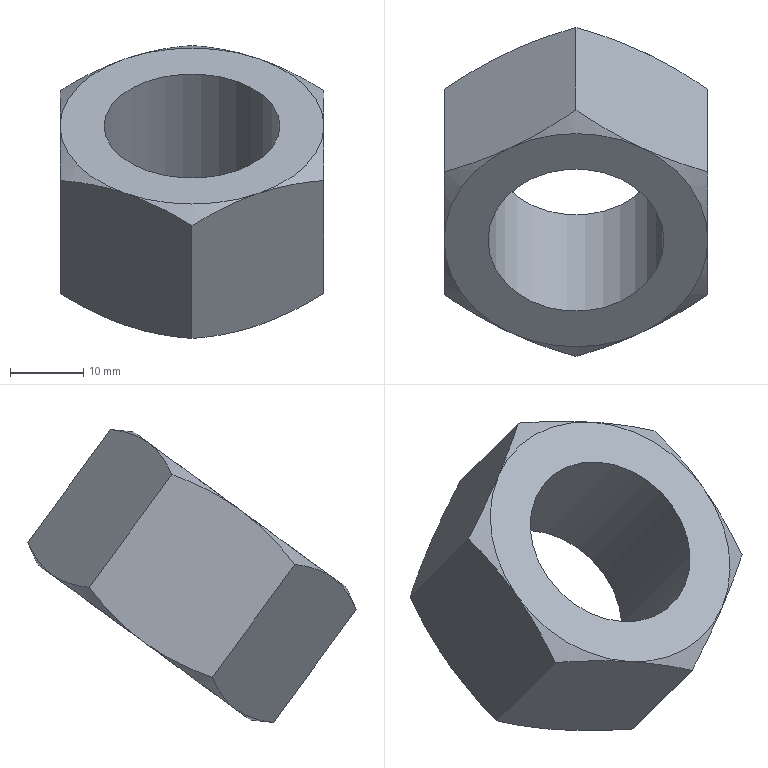Component | SolidWorks | hex nut gradec_iso-10 | 1 solid | 22 faces | box 36 x 44.81 x 39.96 mm | volume 14839 mm3 | cone 12 | plane 8 | cylinder 2 | commonest cylinder face diameters 24 x2
STEP:
#1=COLOUR_RGB('',0.7922,0.8196,0.9333);
#2=FILL_AREA_STYLE_COLOUR('',#1);
#3=FILL_AREA_STYLE('',(#2));
#4=SURFACE_STYLE_FILL_AREA(#3);
#5=SURFACE_SIDE_STYLE('',(#4));
#6=SURFACE_STYLE_USAGE(.BOTH.,#5);
#7=PRESENTATION_STYLE_ASSIGNMENT((#6));
#8=CARTESIAN_POINT('',(-39.394,24.717,14.549));
#9=VERTEX_POINT('',#8);
#10=CARTESIAN_POINT('',(-38.449,24.717,14.549));
#11=VERTEX_POINT('',#10);
#12=CARTESIAN_POINT('',(-38.921,24.717,14.549));
#13=DIRECTION('',(0.,-0.5907,0.8069));
#14=DIRECTION('',(1.,0.,0.));
#15=AXIS2_PLACEMENT_3D('',#12,#13,#14);
#16=CIRCLE('',#15,0.4724);
#17=EDGE_CURVE('',#9,#11,#16,.T.);
#18=ORIENTED_EDGE('',*,*,#17,.F.);
#19=CARTESIAN_POINT('',(-39.394,24.198,15.258));
#20=VERTEX_POINT('',#19);
#21=CARTESIAN_POINT('',(-39.394,24.717,14.549));
#22=DIRECTION('',(0.,-0.5907,0.8069));
#23=VECTOR('',#22,39.37);
#24=LINE('',#21,#23);
#25=EDGE_CURVE('',#9,#20,#24,.T.);
#26=ORIENTED_EDGE('',*,*,#25,.T.);
#27=CARTESIAN_POINT('',(-38.449,24.198,15.258));
#28=VERTEX_POINT('',#27);
#29=CARTESIAN_POINT('',(-38.921,24.198,15.258));
#30=DIRECTION('',(0.,-0.5907,0.8069));
#31=DIRECTION('',(1.,0.,0.));
#32=AXIS2_PLACEMENT_3D('',#29,#30,#31);
#33=CIRCLE('',#32,0.4724);
#34=EDGE_CURVE('',#20,#28,#33,.T.);
#35=ORIENTED_EDGE('',*,*,#34,.T.);
#36=CARTESIAN_POINT('',(-38.449,24.717,14.549));
#37=DIRECTION('',(0.,-0.5907,0.8069));
#38=VECTOR('',#37,39.37);
#39=LINE('',#36,#38);
#40=EDGE_CURVE('',#11,#28,#39,.T.);
#41=ORIENTED_EDGE('',*,*,#40,.F.);
#42=EDGE_LOOP('',(#18,#26,#35,#41));
#43=FACE_OUTER_BOUND('',#42,.T.);
#44=CARTESIAN_POINT('',(-38.921,24.717,14.549));
#45=DIRECTION('',(0.,-0.5907,0.8069));
#46=DIRECTION('',(1.,0.,0.));
#47=AXIS2_PLACEMENT_3D('',#44,#45,#46);
#48=CYLINDRICAL_SURFACE('',#47,0.4724);
#49=ADVANCED_FACE('',(#43),#48,.F.);
#50=CARTESIAN_POINT('',(-39.63,25.01,14.842));
#51=VERTEX_POINT('',#50);
#52=CARTESIAN_POINT('',(-39.63,24.566,15.448));
#53=VERTEX_POINT('',#52);
#54=CARTESIAN_POINT('',(-39.63,25.047,14.791));
#55=DIRECTION('',(0.,-0.5907,0.8069));
#56=VECTOR('',#55,39.37);
#57=LINE('',#54,#56);
#58=EDGE_CURVE('',#51,#53,#57,.T.);
#59=ORIENTED_EDGE('',*,*,#58,.T.);
#60=CARTESIAN_POINT('',(-39.276,24.693,15.62));
#61=VERTEX_POINT('',#60);
#62=CARTESIAN_POINT('',(-39.63,24.566,15.448));
#63=CARTESIAN_POINT('',(-39.572,24.581,15.484));
#64=CARTESIAN_POINT('',(-39.514,24.599,15.517));
#65=CARTESIAN_POINT('',(-39.396,24.641,15.575));
#66=CARTESIAN_POINT('',(-39.336,24.665,15.6));
#67=CARTESIAN_POINT('',(-39.276,24.693,15.62));
#68=B_SPLINE_CURVE_WITH_KNOTS('',3,(#62,#63,#64,#65,#66,#67),.UNSPECIFIED.,.F.,.F.,(4,2,4),(0.00000024,0.005258,0.01052),.UNSPECIFIED.);
#69=EDGE_CURVE('',#53,#61,#68,.T.);
#70=ORIENTED_EDGE('',*,*,#69,.T.);
#71=CARTESIAN_POINT('',(-38.921,24.896,15.69));
#72=VERTEX_POINT('',#71);
#73=CARTESIAN_POINT('',(-39.276,24.693,15.62));
#74=CARTESIAN_POINT('',(-39.261,24.701,15.626));
#75=CARTESIAN_POINT('',(-39.245,24.708,15.63));
#76=CARTESIAN_POINT('',(-39.215,24.723,15.639));
#77=CARTESIAN_POINT('',(-39.2,24.73,15.644));
#78=CARTESIAN_POINT('',(-39.156,24.754,15.655));
#79=CARTESIAN_POINT('',(-39.126,24.77,15.662));
#80=CARTESIAN_POINT('',(-39.037,24.821,15.679));
#81=CARTESIAN_POINT('',(-38.979,24.858,15.686));
#82=CARTESIAN_POINT('',(-38.921,24.896,15.69));
#83=B_SPLINE_CURVE_WITH_KNOTS('',3,(#73,#74,#75,#76,#77,#78,#79,#80,#81,#82),.UNSPECIFIED.,.F.,.F.,(4,2,2,2,4),(0.01052,0.01183,0.01313,0.01575,0.02099),.UNSPECIFIED.);
#84=EDGE_CURVE('',#61,#72,#83,.T.);
#85=ORIENTED_EDGE('',*,*,#84,.T.);
#86=CARTESIAN_POINT('',(-38.921,25.34,15.084));
#87=VERTEX_POINT('',#86);
#88=CARTESIAN_POINT('',(-38.921,25.377,15.033));
#89=DIRECTION('',(0.,-0.5907,0.8069));
#90=VECTOR('',#89,39.37);
#91=LINE('',#88,#90);
#92=EDGE_CURVE('',#87,#72,#91,.T.);
#93=ORIENTED_EDGE('',*,*,#92,.F.);
#94=CARTESIAN_POINT('',(-39.276,25.212,14.912));
#95=VERTEX_POINT('',#94);
#96=CARTESIAN_POINT('',(-39.276,25.212,14.912));
#97=CARTESIAN_POINT('',(-39.261,25.219,14.917));
#98=CARTESIAN_POINT('',(-39.245,25.226,14.923));
#99=CARTESIAN_POINT('',(-39.215,25.239,14.934));
#100=CARTESIAN_POINT('',(-39.2,25.245,14.94));
#101=CARTESIAN_POINT('',(-39.156,25.264,14.959));
#102=CARTESIAN_POINT('',(-39.126,25.275,14.972));
#103=CARTESIAN_POINT('',(-39.037,25.307,15.016));
#104=CARTESIAN_POINT('',(-38.979,25.324,15.049));
#105=CARTESIAN_POINT('',(-38.921,25.34,15.084));
#106=B_SPLINE_CURVE_WITH_KNOTS('',3,(#96,#97,#98,#99,#100,#101,#102,#103,#104,#105),.UNSPECIFIED.,.F.,.F.,(4,2,2,2,4),(0.01052,0.01183,0.01313,0.01575,0.02099),.UNSPECIFIED.);
#107=EDGE_CURVE('',#95,#87,#106,.T.);
#108=ORIENTED_EDGE('',*,*,#107,.F.);
#109=CARTESIAN_POINT('',(-39.63,25.01,14.842));
#110=CARTESIAN_POINT('',(-39.572,25.048,14.846));
#111=CARTESIAN_POINT('',(-39.514,25.085,14.853));
#112=CARTESIAN_POINT('',(-39.396,25.153,14.876));
#113=CARTESIAN_POINT('',(-39.336,25.184,14.891));
#114=CARTESIAN_POINT('',(-39.276,25.212,14.912));
#115=B_SPLINE_CURVE_WITH_KNOTS('',3,(#109,#110,#111,#112,#113,#114),.UNSPECIFIED.,.F.,.F.,(4,2,4),(0.00000024,0.005258,0.01052),.UNSPECIFIED.);
#116=EDGE_CURVE('',#51,#95,#115,.T.);
#117=ORIENTED_EDGE('',*,*,#116,.F.);
#118=EDGE_LOOP('',(#59,#70,#85,#93,#108,#117));
#119=FACE_OUTER_BOUND('',#118,.T.);
#120=CARTESIAN_POINT('',(-38.921,25.377,15.033));
#121=DIRECTION('',(-0.5,0.6988,0.5116));
#122=DIRECTION('',(-0.866,-0.4034,-0.2954));
#123=AXIS2_PLACEMENT_3D('',#120,#121,#122);
#124=PLANE('',#123);
#125=ADVANCED_FACE('',(#119),#124,.T.);
#126=ORIENTED_EDGE('',*,*,#92,.T.);
#127=CARTESIAN_POINT('',(-38.567,24.693,15.62));
#128=VERTEX_POINT('',#127);
#129=CARTESIAN_POINT('',(-38.921,24.896,15.69));
#130=CARTESIAN_POINT('',(-38.863,24.858,15.686));
#131=CARTESIAN_POINT('',(-38.805,24.821,15.679));
#132=CARTESIAN_POINT('',(-38.687,24.753,15.656));
#133=CARTESIAN_POINT('',(-38.627,24.722,15.641));
#134=CARTESIAN_POINT('',(-38.567,24.693,15.62));
#135=B_SPLINE_CURVE_WITH_KNOTS('',3,(#129,#130,#131,#132,#133,#134),.UNSPECIFIED.,.F.,.F.,(4,2,4),(0.00000024,0.005258,0.01052),.UNSPECIFIED.);
#136=EDGE_CURVE('',#72,#128,#135,.T.);
#137=ORIENTED_EDGE('',*,*,#136,.T.);
#138=CARTESIAN_POINT('',(-38.213,24.566,15.448));
#139=VERTEX_POINT('',#138);
#140=CARTESIAN_POINT('',(-38.567,24.693,15.62));
#141=CARTESIAN_POINT('',(-38.552,24.686,15.615));
#142=CARTESIAN_POINT('',(-38.537,24.68,15.61));
#143=CARTESIAN_POINT('',(-38.507,24.667,15.598));
#144=CARTESIAN_POINT('',(-38.492,24.66,15.592));
#145=CARTESIAN_POINT('',(-38.447,24.642,15.574));
#146=CARTESIAN_POINT('',(-38.417,24.631,15.56));
#147=CARTESIAN_POINT('',(-38.329,24.599,15.516));
#148=CARTESIAN_POINT('',(-38.27,24.581,15.484));
#149=CARTESIAN_POINT('',(-38.213,24.566,15.448));
#150=B_SPLINE_CURVE_WITH_KNOTS('',3,(#140,#141,#142,#143,#144,#145,#146,#147,#148,#149),.UNSPECIFIED.,.F.,.F.,(4,2,2,2,4),(0.01052,0.01183,0.01313,0.01575,0.02099),.UNSPECIFIED.);
#151=EDGE_CURVE('',#128,#139,#150,.T.);
#152=ORIENTED_EDGE('',*,*,#151,.T.);
#153=CARTESIAN_POINT('',(-38.213,25.01,14.842));
#154=VERTEX_POINT('',#153);
#155=CARTESIAN_POINT('',(-38.213,25.047,14.791));
#156=DIRECTION('',(0.,-0.5907,0.8069));
#157=VECTOR('',#156,39.37);
#158=LINE('',#155,#157);
#159=EDGE_CURVE('',#154,#139,#158,.T.);
#160=ORIENTED_EDGE('',*,*,#159,.F.);
#161=CARTESIAN_POINT('',(-38.567,25.212,14.912));
#162=VERTEX_POINT('',#161);
#163=CARTESIAN_POINT('',(-38.567,25.212,14.912));
#164=CARTESIAN_POINT('',(-38.552,25.205,14.907));
#165=CARTESIAN_POINT('',(-38.537,25.198,14.902));
#166=CARTESIAN_POINT('',(-38.507,25.183,14.893));
#167=CARTESIAN_POINT('',(-38.492,25.175,14.889));
#168=CARTESIAN_POINT('',(-38.447,25.152,14.877));
#169=CARTESIAN_POINT('',(-38.417,25.136,14.87));
#170=CARTESIAN_POINT('',(-38.329,25.085,14.853));
#171=CARTESIAN_POINT('',(-38.27,25.048,14.846));
#172=CARTESIAN_POINT('',(-38.213,25.01,14.842));
#173=B_SPLINE_CURVE_WITH_KNOTS('',3,(#163,#164,#165,#166,#167,#168,#169,#170,#171,#172),.UNSPECIFIED.,.F.,.F.,(4,2,2,2,4),(0.01052,0.01183,0.01313,0.01575,0.02099),.UNSPECIFIED.);
#174=EDGE_CURVE('',#162,#154,#173,.T.);
#175=ORIENTED_EDGE('',*,*,#174,.F.);
#176=CARTESIAN_POINT('',(-38.921,25.34,15.084));
#177=CARTESIAN_POINT('',(-38.863,25.324,15.049));
#178=CARTESIAN_POINT('',(-38.805,25.306,15.016));
#179=CARTESIAN_POINT('',(-38.687,25.264,14.958));
#180=CARTESIAN_POINT('',(-38.627,25.24,14.933));
#181=CARTESIAN_POINT('',(-38.567,25.212,14.912));
#182=B_SPLINE_CURVE_WITH_KNOTS('',3,(#176,#177,#178,#179,#180,#181),.UNSPECIFIED.,.F.,.F.,(4,2,4),(0.00000024,0.005258,0.01052),.UNSPECIFIED.);
#183=EDGE_CURVE('',#87,#162,#182,.T.);
#184=ORIENTED_EDGE('',*,*,#183,.F.);
#185=EDGE_LOOP('',(#126,#137,#152,#160,#175,#184));
#186=FACE_OUTER_BOUND('',#185,.T.);
#187=CARTESIAN_POINT('',(-38.213,25.047,14.791));
#188=DIRECTION('',(0.5,0.6988,0.5116));
#189=DIRECTION('',(-0.866,0.4034,0.2954));
#190=AXIS2_PLACEMENT_3D('',#187,#188,#189);
#191=PLANE('',#190);
#192=ADVANCED_FACE('',(#186),#191,.T.);
#193=CARTESIAN_POINT('',(-38.213,23.906,14.965));
#194=VERTEX_POINT('',#193);
#195=CARTESIAN_POINT('',(-38.213,24.198,15.258));
#196=VERTEX_POINT('',#195);
#197=CARTESIAN_POINT('',(-38.213,23.906,14.965));
#198=CARTESIAN_POINT('',(-38.213,23.927,14.992));
#199=CARTESIAN_POINT('',(-38.213,23.949,15.019));
#200=CARTESIAN_POINT('',(-38.213,23.994,15.072));
#201=CARTESIAN_POINT('',(-38.213,24.018,15.098));
#202=CARTESIAN_POINT('',(-38.213,24.091,15.172));
#203=CARTESIAN_POINT('',(-38.213,24.143,15.217));
#204=CARTESIAN_POINT('',(-38.213,24.198,15.258));
#205=B_SPLINE_CURVE_WITH_KNOTS('',3,(#197,#198,#199,#200,#201,#202,#203,#204),.UNSPECIFIED.,.F.,.F.,(4,2,2,4),(0.01854,0.02117,0.0238,0.02905),.UNSPECIFIED.);
#206=EDGE_CURVE('',#194,#196,#205,.T.);
#207=ORIENTED_EDGE('',*,*,#206,.F.);
#208=CARTESIAN_POINT('',(-38.213,24.349,14.359));
#209=VERTEX_POINT('',#208);
#210=CARTESIAN_POINT('',(-38.213,24.387,14.308));
#211=DIRECTION('',(0.,-0.5907,0.8069));
#212=VECTOR('',#211,39.37);
#213=LINE('',#210,#212);
#214=EDGE_CURVE('',#209,#194,#213,.T.);
#215=ORIENTED_EDGE('',*,*,#214,.F.);
#216=CARTESIAN_POINT('',(-38.213,24.717,14.549));
#217=VERTEX_POINT('',#216);
#218=CARTESIAN_POINT('',(-38.213,24.349,14.359));
#219=CARTESIAN_POINT('',(-38.213,24.382,14.371));
#220=CARTESIAN_POINT('',(-38.213,24.414,14.383));
#221=CARTESIAN_POINT('',(-38.213,24.478,14.411));
#222=CARTESIAN_POINT('',(-38.213,24.51,14.426));
#223=CARTESIAN_POINT('',(-38.213,24.602,14.473));
#224=CARTESIAN_POINT('',(-38.213,24.661,14.509));
#225=CARTESIAN_POINT('',(-38.213,24.717,14.549));
#226=B_SPLINE_CURVE_WITH_KNOTS('',3,(#218,#219,#220,#221,#222,#223,#224,#225),.UNSPECIFIED.,.F.,.F.,(4,2,2,4),(0.01854,0.02117,0.0238,0.02905),.UNSPECIFIED.);
#227=EDGE_CURVE('',#209,#217,#226,.T.);
#228=ORIENTED_EDGE('',*,*,#227,.T.);
#229=CARTESIAN_POINT('',(-38.213,24.717,14.549));
#230=CARTESIAN_POINT('',(-38.213,24.745,14.57));
#231=CARTESIAN_POINT('',(-38.213,24.772,14.592));
#232=CARTESIAN_POINT('',(-38.213,24.825,14.637));
#233=CARTESIAN_POINT('',(-38.213,24.85,14.661));
#234=CARTESIAN_POINT('',(-38.213,24.923,14.735));
#235=CARTESIAN_POINT('',(-38.213,24.968,14.788));
#236=CARTESIAN_POINT('',(-38.213,25.01,14.842));
#237=B_SPLINE_CURVE_WITH_KNOTS('',3,(#229,#230,#231,#232,#233,#234,#235,#236),.UNSPECIFIED.,.F.,.F.,(4,2,2,4),(0.02905,0.03168,0.03431,0.03957),.UNSPECIFIED.);
#238=EDGE_CURVE('',#217,#154,#237,.T.);
#239=ORIENTED_EDGE('',*,*,#238,.T.);
#240=ORIENTED_EDGE('',*,*,#159,.T.);
#241=CARTESIAN_POINT('',(-38.213,24.198,15.258));
#242=CARTESIAN_POINT('',(-38.213,24.226,15.278));
#243=CARTESIAN_POINT('',(-38.213,24.255,15.298));
#244=CARTESIAN_POINT('',(-38.213,24.315,15.334));
#245=CARTESIAN_POINT('',(-38.213,24.345,15.351));
#246=CARTESIAN_POINT('',(-38.213,24.438,15.398));
#247=CARTESIAN_POINT('',(-38.213,24.501,15.425));
#248=CARTESIAN_POINT('',(-38.213,24.566,15.448));
#249=B_SPLINE_CURVE_WITH_KNOTS('',3,(#241,#242,#243,#244,#245,#246,#247,#248),.UNSPECIFIED.,.F.,.F.,(4,2,2,4),(0.02905,0.03168,0.03431,0.03957),.UNSPECIFIED.);
#250=EDGE_CURVE('',#196,#139,#249,.T.);
#251=ORIENTED_EDGE('',*,*,#250,.F.);
#252=EDGE_LOOP('',(#207,#215,#228,#239,#240,#251));
#253=FACE_OUTER_BOUND('',#252,.T.);
#254=CARTESIAN_POINT('',(-38.213,25.047,14.791));
#255=DIRECTION('',(-1.,-0.,-0.));
#256=DIRECTION('',(0.,-0.5907,0.8069));
#257=AXIS2_PLACEMENT_3D('',#254,#255,#256);
#258=PLANE('',#257);
#259=ADVANCED_FACE('',(#253),#258,.F.);
#260=ORIENTED_EDGE('',*,*,#214,.T.);
#261=CARTESIAN_POINT('',(-38.567,23.703,14.895));
#262=VERTEX_POINT('',#261);
#263=CARTESIAN_POINT('',(-38.213,23.906,14.965));
#264=CARTESIAN_POINT('',(-38.271,23.867,14.961));
#265=CARTESIAN_POINT('',(-38.329,23.831,14.954));
#266=CARTESIAN_POINT('',(-38.447,23.763,14.931));
#267=CARTESIAN_POINT('',(-38.507,23.731,14.916));
#268=CARTESIAN_POINT('',(-38.567,23.703,14.895));
#269=B_SPLINE_CURVE_WITH_KNOTS('',3,(#263,#264,#265,#266,#267,#268),.UNSPECIFIED.,.F.,.F.,(4,2,4),(0.00000024,0.005258,0.01052),.UNSPECIFIED.);
#270=EDGE_CURVE('',#194,#262,#269,.T.);
#271=ORIENTED_EDGE('',*,*,#270,.T.);
#272=CARTESIAN_POINT('',(-38.921,23.575,14.723));
#273=VERTEX_POINT('',#272);
#274=CARTESIAN_POINT('',(-38.567,23.703,14.895));
#275=CARTESIAN_POINT('',(-38.582,23.696,14.89));
#276=CARTESIAN_POINT('',(-38.597,23.689,14.885));
#277=CARTESIAN_POINT('',(-38.627,23.676,14.873));
#278=CARTESIAN_POINT('',(-38.642,23.67,14.867));
#279=CARTESIAN_POINT('',(-38.687,23.652,14.848));
#280=CARTESIAN_POINT('',(-38.717,23.64,14.835));
#281=CARTESIAN_POINT('',(-38.805,23.609,14.791));
#282=CARTESIAN_POINT('',(-38.863,23.591,14.759));
#283=CARTESIAN_POINT('',(-38.921,23.575,14.723));
#284=B_SPLINE_CURVE_WITH_KNOTS('',3,(#274,#275,#276,#277,#278,#279,#280,#281,#282,#283),.UNSPECIFIED.,.F.,.F.,(4,2,2,2,4),(0.01052,0.01183,0.01313,0.01575,0.02099),.UNSPECIFIED.);
#285=EDGE_CURVE('',#262,#273,#284,.T.);
#286=ORIENTED_EDGE('',*,*,#285,.T.);
#287=CARTESIAN_POINT('',(-38.921,24.019,14.117));
#288=VERTEX_POINT('',#287);
#289=CARTESIAN_POINT('',(-38.921,24.057,14.066));
#290=DIRECTION('',(0.,-0.5907,0.8069));
#291=VECTOR('',#290,39.37);
#292=LINE('',#289,#291);
#293=EDGE_CURVE('',#288,#273,#292,.T.);
#294=ORIENTED_EDGE('',*,*,#293,.F.);
#295=CARTESIAN_POINT('',(-38.567,24.222,14.187));
#296=VERTEX_POINT('',#295);
#297=CARTESIAN_POINT('',(-38.567,24.222,14.187));
#298=CARTESIAN_POINT('',(-38.582,24.215,14.182));
#299=CARTESIAN_POINT('',(-38.597,24.208,14.177));
#300=CARTESIAN_POINT('',(-38.627,24.193,14.168));
#301=CARTESIAN_POINT('',(-38.642,24.185,14.164));
#302=CARTESIAN_POINT('',(-38.687,24.162,14.152));
#303=CARTESIAN_POINT('',(-38.717,24.145,14.145));
#304=CARTESIAN_POINT('',(-38.805,24.094,14.128));
#305=CARTESIAN_POINT('',(-38.863,24.058,14.121));
#306=CARTESIAN_POINT('',(-38.921,24.019,14.117));
#307=B_SPLINE_CURVE_WITH_KNOTS('',3,(#297,#298,#299,#300,#301,#302,#303,#304,#305,#306),.UNSPECIFIED.,.F.,.F.,(4,2,2,2,4),(0.01052,0.01183,0.01313,0.01575,0.02099),.UNSPECIFIED.);
#308=EDGE_CURVE('',#296,#288,#307,.T.);
#309=ORIENTED_EDGE('',*,*,#308,.F.);
#310=CARTESIAN_POINT('',(-38.213,24.349,14.359));
#311=CARTESIAN_POINT('',(-38.271,24.334,14.323));
#312=CARTESIAN_POINT('',(-38.329,24.316,14.291));
#313=CARTESIAN_POINT('',(-38.447,24.274,14.233));
#314=CARTESIAN_POINT('',(-38.507,24.25,14.207));
#315=CARTESIAN_POINT('',(-38.567,24.222,14.187));
#316=B_SPLINE_CURVE_WITH_KNOTS('',3,(#310,#311,#312,#313,#314,#315),.UNSPECIFIED.,.F.,.F.,(4,2,4),(0.00000024,0.005258,0.01052),.UNSPECIFIED.);
#317=EDGE_CURVE('',#209,#296,#316,.T.);
#318=ORIENTED_EDGE('',*,*,#317,.F.);
#319=EDGE_LOOP('',(#260,#271,#286,#294,#309,#318));
#320=FACE_OUTER_BOUND('',#319,.T.);
#321=CARTESIAN_POINT('',(-38.921,24.057,14.066));
#322=DIRECTION('',(0.5,-0.6988,-0.5116));
#323=DIRECTION('',(0.866,0.4034,0.2954));
#324=AXIS2_PLACEMENT_3D('',#321,#322,#323);
#325=PLANE('',#324);
#326=ADVANCED_FACE('',(#320),#325,.T.);
#327=ORIENTED_EDGE('',*,*,#293,.T.);
#328=CARTESIAN_POINT('',(-39.276,23.703,14.895));
#329=VERTEX_POINT('',#328);
#330=CARTESIAN_POINT('',(-38.921,23.575,14.723));
#331=CARTESIAN_POINT('',(-38.979,23.591,14.759));
#332=CARTESIAN_POINT('',(-39.038,23.609,14.791));
#333=CARTESIAN_POINT('',(-39.156,23.651,14.849));
#334=CARTESIAN_POINT('',(-39.215,23.675,14.875));
#335=CARTESIAN_POINT('',(-39.276,23.703,14.895));
#336=B_SPLINE_CURVE_WITH_KNOTS('',3,(#330,#331,#332,#333,#334,#335),.UNSPECIFIED.,.F.,.F.,(4,2,4),(0.00000024,0.005258,0.01052),.UNSPECIFIED.);
#337=EDGE_CURVE('',#273,#329,#336,.T.);
#338=ORIENTED_EDGE('',*,*,#337,.T.);
#339=CARTESIAN_POINT('',(-39.63,23.906,14.965));
#340=VERTEX_POINT('',#339);
#341=CARTESIAN_POINT('',(-39.276,23.703,14.895));
#342=CARTESIAN_POINT('',(-39.291,23.71,14.9));
#343=CARTESIAN_POINT('',(-39.306,23.717,14.905));
#344=CARTESIAN_POINT('',(-39.336,23.732,14.914));
#345=CARTESIAN_POINT('',(-39.351,23.74,14.919));
#346=CARTESIAN_POINT('',(-39.396,23.763,14.93));
#347=CARTESIAN_POINT('',(-39.425,23.78,14.937));
#348=CARTESIAN_POINT('',(-39.514,23.831,14.954));
#349=CARTESIAN_POINT('',(-39.572,23.867,14.961));
#350=CARTESIAN_POINT('',(-39.63,23.906,14.965));
#351=B_SPLINE_CURVE_WITH_KNOTS('',3,(#341,#342,#343,#344,#345,#346,#347,#348,#349,#350),.UNSPECIFIED.,.F.,.F.,(4,2,2,2,4),(0.01052,0.01183,0.01313,0.01575,0.02099),.UNSPECIFIED.);
#352=EDGE_CURVE('',#329,#340,#351,.T.);
#353=ORIENTED_EDGE('',*,*,#352,.T.);
#354=CARTESIAN_POINT('',(-39.63,24.349,14.359));
#355=VERTEX_POINT('',#354);
#356=CARTESIAN_POINT('',(-39.63,24.387,14.308));
#357=DIRECTION('',(0.,-0.5907,0.8069));
#358=VECTOR('',#357,39.37);
#359=LINE('',#356,#358);
#360=EDGE_CURVE('',#355,#340,#359,.T.);
#361=ORIENTED_EDGE('',*,*,#360,.F.);
#362=CARTESIAN_POINT('',(-39.276,24.222,14.187));
#363=VERTEX_POINT('',#362);
#364=CARTESIAN_POINT('',(-39.276,24.222,14.187));
#365=CARTESIAN_POINT('',(-39.291,24.229,14.192));
#366=CARTESIAN_POINT('',(-39.306,24.236,14.197));
#367=CARTESIAN_POINT('',(-39.336,24.249,14.209));
#368=CARTESIAN_POINT('',(-39.351,24.255,14.215));
#369=CARTESIAN_POINT('',(-39.396,24.273,14.234));
#370=CARTESIAN_POINT('',(-39.425,24.285,14.247));
#371=CARTESIAN_POINT('',(-39.514,24.316,14.291));
#372=CARTESIAN_POINT('',(-39.572,24.334,14.324));
#373=CARTESIAN_POINT('',(-39.63,24.349,14.359));
#374=B_SPLINE_CURVE_WITH_KNOTS('',3,(#364,#365,#366,#367,#368,#369,#370,#371,#372,#373),.UNSPECIFIED.,.F.,.F.,(4,2,2,2,4),(0.01052,0.01183,0.01313,0.01575,0.02099),.UNSPECIFIED.);
#375=EDGE_CURVE('',#363,#355,#374,.T.);
#376=ORIENTED_EDGE('',*,*,#375,.F.);
#377=CARTESIAN_POINT('',(-38.921,24.019,14.117));
#378=CARTESIAN_POINT('',(-38.979,24.058,14.121));
#379=CARTESIAN_POINT('',(-39.038,24.094,14.128));
#380=CARTESIAN_POINT('',(-39.156,24.162,14.151));
#381=CARTESIAN_POINT('',(-39.215,24.194,14.166));
#382=CARTESIAN_POINT('',(-39.276,24.222,14.187));
#383=B_SPLINE_CURVE_WITH_KNOTS('',3,(#377,#378,#379,#380,#381,#382),.UNSPECIFIED.,.F.,.F.,(4,2,4),(0.00000024,0.005258,0.01052),.UNSPECIFIED.);
#384=EDGE_CURVE('',#288,#363,#383,.T.);
#385=ORIENTED_EDGE('',*,*,#384,.F.);
#386=EDGE_LOOP('',(#327,#338,#353,#361,#376,#385));
#387=FACE_OUTER_BOUND('',#386,.T.);
#388=CARTESIAN_POINT('',(-39.63,24.387,14.308));
#389=DIRECTION('',(-0.5,-0.6988,-0.5116));
#390=DIRECTION('',(0.866,-0.4034,-0.2954));
#391=AXIS2_PLACEMENT_3D('',#388,#389,#390);
#392=PLANE('',#391);
#393=ADVANCED_FACE('',(#387),#392,.T.);
#394=ORIENTED_EDGE('',*,*,#360,.T.);
#395=CARTESIAN_POINT('',(-39.63,24.198,15.258));
#396=VERTEX_POINT('',#395);
#397=CARTESIAN_POINT('',(-39.63,23.906,14.965));
#398=CARTESIAN_POINT('',(-39.63,23.927,14.992));
#399=CARTESIAN_POINT('',(-39.63,23.949,15.019));
#400=CARTESIAN_POINT('',(-39.63,23.994,15.072));
#401=CARTESIAN_POINT('',(-39.63,24.018,15.098));
#402=CARTESIAN_POINT('',(-39.63,24.091,15.172));
#403=CARTESIAN_POINT('',(-39.63,24.143,15.217));
#404=CARTESIAN_POINT('',(-39.63,24.198,15.258));
#405=B_SPLINE_CURVE_WITH_KNOTS('',3,(#397,#398,#399,#400,#401,#402,#403,#404),.UNSPECIFIED.,.F.,.F.,(4,2,2,4),(0.01854,0.02117,0.0238,0.02905),.UNSPECIFIED.);
#406=EDGE_CURVE('',#340,#396,#405,.T.);
#407=ORIENTED_EDGE('',*,*,#406,.T.);
#408=CARTESIAN_POINT('',(-39.63,24.198,15.258));
#409=CARTESIAN_POINT('',(-39.63,24.226,15.278));
#410=CARTESIAN_POINT('',(-39.63,24.255,15.298));
#411=CARTESIAN_POINT('',(-39.63,24.315,15.334));
#412=CARTESIAN_POINT('',(-39.63,24.345,15.351));
#413=CARTESIAN_POINT('',(-39.63,24.438,15.398));
#414=CARTESIAN_POINT('',(-39.63,24.501,15.425));
#415=CARTESIAN_POINT('',(-39.63,24.566,15.448));
#416=B_SPLINE_CURVE_WITH_KNOTS('',3,(#408,#409,#410,#411,#412,#413,#414,#415),.UNSPECIFIED.,.F.,.F.,(4,2,2,4),(0.02905,0.03168,0.03431,0.03957),.UNSPECIFIED.);
#417=EDGE_CURVE('',#396,#53,#416,.T.);
#418=ORIENTED_EDGE('',*,*,#417,.T.);
#419=ORIENTED_EDGE('',*,*,#58,.F.);
#420=CARTESIAN_POINT('',(-39.63,24.717,14.549));
#421=VERTEX_POINT('',#420);
#422=CARTESIAN_POINT('',(-39.63,24.717,14.549));
#423=CARTESIAN_POINT('',(-39.63,24.745,14.57));
#424=CARTESIAN_POINT('',(-39.63,24.772,14.592));
#425=CARTESIAN_POINT('',(-39.63,24.825,14.637));
#426=CARTESIAN_POINT('',(-39.63,24.85,14.661));
#427=CARTESIAN_POINT('',(-39.63,24.923,14.735));
#428=CARTESIAN_POINT('',(-39.63,24.968,14.788));
#429=CARTESIAN_POINT('',(-39.63,25.01,14.842));
#430=B_SPLINE_CURVE_WITH_KNOTS('',3,(#422,#423,#424,#425,#426,#427,#428,#429),.UNSPECIFIED.,.F.,.F.,(4,2,2,4),(0.02905,0.03168,0.03431,0.03957),.UNSPECIFIED.);
#431=EDGE_CURVE('',#421,#51,#430,.T.);
#432=ORIENTED_EDGE('',*,*,#431,.F.);
#433=CARTESIAN_POINT('',(-39.63,24.349,14.359));
#434=CARTESIAN_POINT('',(-39.63,24.382,14.371));
#435=CARTESIAN_POINT('',(-39.63,24.414,14.383));
#436=CARTESIAN_POINT('',(-39.63,24.478,14.411));
#437=CARTESIAN_POINT('',(-39.63,24.51,14.426));
#438=CARTESIAN_POINT('',(-39.63,24.602,14.473));
#439=CARTESIAN_POINT('',(-39.63,24.661,14.509));
#440=CARTESIAN_POINT('',(-39.63,24.717,14.549));
#441=B_SPLINE_CURVE_WITH_KNOTS('',3,(#433,#434,#435,#436,#437,#438,#439,#440),.UNSPECIFIED.,.F.,.F.,(4,2,2,4),(0.01854,0.02117,0.0238,0.02905),.UNSPECIFIED.);
#442=EDGE_CURVE('',#355,#421,#441,.T.);
#443=ORIENTED_EDGE('',*,*,#442,.F.);
#444=EDGE_LOOP('',(#394,#407,#418,#419,#432,#443));
#445=FACE_OUTER_BOUND('',#444,.T.);
#446=CARTESIAN_POINT('',(-39.63,25.047,14.791));
#447=DIRECTION('',(-1.,-0.,-0.));
#448=DIRECTION('',(0.,-0.5907,0.8069));
#449=AXIS2_PLACEMENT_3D('',#446,#447,#448);
#450=PLANE('',#449);
#451=ADVANCED_FACE('',(#445),#450,.T.);
#452=CARTESIAN_POINT('',(-38.921,24.198,15.258));
#453=DIRECTION('',(0.,-0.5907,0.8069));
#454=DIRECTION('',(1.,0.,0.));
#455=AXIS2_PLACEMENT_3D('',#452,#453,#454);
#456=CIRCLE('',#455,0.4724);
#457=EDGE_CURVE('',#28,#20,#456,.T.);
#458=ORIENTED_EDGE('',*,*,#457,.F.);
#459=ORIENTED_EDGE('',*,*,#34,.F.);
#460=EDGE_LOOP('',(#458,#459));
#461=FACE_BOUND('',#460,.T.);
#462=CARTESIAN_POINT('',(-38.921,24.198,15.258));
#463=DIRECTION('',(-0.,0.5907,-0.8069));
#464=DIRECTION('',(-1.,0.,0.));
#465=AXIS2_PLACEMENT_3D('',#462,#463,#464);
#466=CIRCLE('',#465,0.7087);
#467=EDGE_CURVE('',#396,#61,#466,.T.);
#468=ORIENTED_EDGE('',*,*,#467,.F.);
#469=CARTESIAN_POINT('',(-38.921,24.198,15.258));
#470=DIRECTION('',(-0.,0.5907,-0.8069));
#471=DIRECTION('',(-1.,0.,0.));
#472=AXIS2_PLACEMENT_3D('',#469,#470,#471);
#473=CIRCLE('',#472,0.7087);
#474=EDGE_CURVE('',#329,#396,#473,.T.);
#475=ORIENTED_EDGE('',*,*,#474,.F.);
#476=CARTESIAN_POINT('',(-38.921,24.198,15.258));
#477=DIRECTION('',(-0.,0.5907,-0.8069));
#478=DIRECTION('',(-1.,0.,0.));
#479=AXIS2_PLACEMENT_3D('',#476,#477,#478);
#480=CIRCLE('',#479,0.7087);
#481=EDGE_CURVE('',#262,#329,#480,.T.);
#482=ORIENTED_EDGE('',*,*,#481,.F.);
#483=CARTESIAN_POINT('',(-38.921,24.198,15.258));
#484=DIRECTION('',(-0.,0.5907,-0.8069));
#485=DIRECTION('',(-1.,0.,0.));
#486=AXIS2_PLACEMENT_3D('',#483,#484,#485);
#487=CIRCLE('',#486,0.7087);
#488=EDGE_CURVE('',#196,#262,#487,.T.);
#489=ORIENTED_EDGE('',*,*,#488,.F.);
#490=CARTESIAN_POINT('',(-38.921,24.198,15.258));
#491=DIRECTION('',(0.,-0.5907,0.8069));
#492=DIRECTION('',(1.,0.,0.));
#493=AXIS2_PLACEMENT_3D('',#490,#491,#492);
#494=CIRCLE('',#493,0.7087);
#495=EDGE_CURVE('',#196,#128,#494,.T.);
#496=ORIENTED_EDGE('',*,*,#495,.T.);
#497=CARTESIAN_POINT('',(-38.921,24.198,15.258));
#498=DIRECTION('',(-0.,0.5907,-0.8069));
#499=DIRECTION('',(-1.,0.,0.));
#500=AXIS2_PLACEMENT_3D('',#497,#498,#499);
#501=CIRCLE('',#500,0.7087);
#502=EDGE_CURVE('',#61,#128,#501,.T.);
#503=ORIENTED_EDGE('',*,*,#502,.F.);
#504=EDGE_LOOP('',(#468,#475,#482,#489,#496,#503));
#505=FACE_OUTER_BOUND('',#504,.T.);
#506=CARTESIAN_POINT('',(-38.921,24.859,15.741));
#507=DIRECTION('',(-0.,0.5907,-0.8069));
#508=DIRECTION('',(-1.,-0.,-0.));
#509=AXIS2_PLACEMENT_3D('',#506,#507,#508);
#510=PLANE('',#509);
#511=ADVANCED_FACE('',(#461,#505),#510,.F.);
#512=CARTESIAN_POINT('',(-38.921,24.717,14.549));
#513=DIRECTION('',(0.,-0.5907,0.8069));
#514=DIRECTION('',(1.,0.,0.));
#515=AXIS2_PLACEMENT_3D('',#512,#513,#514);
#516=CIRCLE('',#515,0.4724);
#517=EDGE_CURVE('',#11,#9,#516,.T.);
#518=ORIENTED_EDGE('',*,*,#517,.T.);
#519=ORIENTED_EDGE('',*,*,#17,.T.);
#520=EDGE_LOOP('',(#518,#519));
#521=FACE_BOUND('',#520,.T.);
#522=CARTESIAN_POINT('',(-38.921,24.717,14.549));
#523=DIRECTION('',(0.,-0.5907,0.8069));
#524=DIRECTION('',(-1.,0.,0.));
#525=AXIS2_PLACEMENT_3D('',#522,#523,#524);
#526=CIRCLE('',#525,0.7087);
#527=EDGE_CURVE('',#421,#363,#526,.T.);
#528=ORIENTED_EDGE('',*,*,#527,.F.);
#529=CARTESIAN_POINT('',(-38.921,24.717,14.549));
#530=DIRECTION('',(0.,-0.5907,0.8069));
#531=DIRECTION('',(-1.,0.,0.));
#532=AXIS2_PLACEMENT_3D('',#529,#530,#531);
#533=CIRCLE('',#532,0.7087);
#534=EDGE_CURVE('',#95,#421,#533,.T.);
#535=ORIENTED_EDGE('',*,*,#534,.F.);
#536=CARTESIAN_POINT('',(-38.921,24.717,14.549));
#537=DIRECTION('',(0.,-0.5907,0.8069));
#538=DIRECTION('',(-1.,-0.,-0.));
#539=AXIS2_PLACEMENT_3D('',#536,#537,#538);
#540=CIRCLE('',#539,0.7087);
#541=EDGE_CURVE('',#162,#95,#540,.T.);
#542=ORIENTED_EDGE('',*,*,#541,.F.);
#543=CARTESIAN_POINT('',(-38.921,24.717,14.549));
#544=DIRECTION('',(0.,-0.5907,0.8069));
#545=DIRECTION('',(1.,0.,0.));
#546=AXIS2_PLACEMENT_3D('',#543,#544,#545);
#547=CIRCLE('',#546,0.7087);
#548=EDGE_CURVE('',#217,#162,#547,.T.);
#549=ORIENTED_EDGE('',*,*,#548,.F.);
#550=CARTESIAN_POINT('',(-38.921,24.717,14.549));
#551=DIRECTION('',(0.,-0.5907,0.8069));
#552=DIRECTION('',(-1.,0.,0.));
#553=AXIS2_PLACEMENT_3D('',#550,#551,#552);
#554=CIRCLE('',#553,0.7087);
#555=EDGE_CURVE('',#296,#217,#554,.T.);
#556=ORIENTED_EDGE('',*,*,#555,.F.);
#557=CARTESIAN_POINT('',(-38.921,24.717,14.549));
#558=DIRECTION('',(0.,-0.5907,0.8069));
#559=DIRECTION('',(-1.,0.,0.));
#560=AXIS2_PLACEMENT_3D('',#557,#558,#559);
#561=CIRCLE('',#560,0.7087);
#562=EDGE_CURVE('',#363,#296,#561,.T.);
#563=ORIENTED_EDGE('',*,*,#562,.F.);
#564=EDGE_LOOP('',(#528,#535,#542,#549,#556,#563));
#565=FACE_OUTER_BOUND('',#564,.T.);
#566=CARTESIAN_POINT('',(-38.921,25.377,15.033));
#567=DIRECTION('',(-0.,0.5907,-0.8069));
#568=DIRECTION('',(-1.,-0.,-0.));
#569=AXIS2_PLACEMENT_3D('',#566,#567,#568);
#570=PLANE('',#569);
#571=ADVANCED_FACE('',(#521,#565),#570,.T.);
#572=ORIENTED_EDGE('',*,*,#25,.F.);
#573=ORIENTED_EDGE('',*,*,#517,.F.);
#574=ORIENTED_EDGE('',*,*,#40,.T.);
#575=ORIENTED_EDGE('',*,*,#457,.T.);
#576=EDGE_LOOP('',(#572,#573,#574,#575));
#577=FACE_OUTER_BOUND('',#576,.T.);
#578=CARTESIAN_POINT('',(-38.921,24.717,14.549));
#579=DIRECTION('',(0.,-0.5907,0.8069));
#580=DIRECTION('',(1.,0.,0.));
#581=AXIS2_PLACEMENT_3D('',#578,#579,#580);
#582=CYLINDRICAL_SURFACE('',#581,0.4724);
#583=ADVANCED_FACE('',(#577),#582,.F.);
#584=ORIENTED_EDGE('',*,*,#116,.T.);
#585=ORIENTED_EDGE('',*,*,#534,.T.);
#586=ORIENTED_EDGE('',*,*,#431,.T.);
#587=EDGE_LOOP('',(#584,#585,#586));
#588=FACE_OUTER_BOUND('',#587,.T.);
#589=CARTESIAN_POINT('',(-38.921,24.717,14.549));
#590=DIRECTION('',(0.,-0.5907,0.8069));
#591=DIRECTION('',(1.,0.,0.));
#592=AXIS2_PLACEMENT_3D('',#589,#590,#591);
#593=CONICAL_SURFACE('',#592,0.7087,1.047);
#594=ADVANCED_FACE('',(#588),#593,.T.);
#595=ORIENTED_EDGE('',*,*,#107,.T.);
#596=ORIENTED_EDGE('',*,*,#183,.T.);
#597=ORIENTED_EDGE('',*,*,#541,.T.);
#598=EDGE_LOOP('',(#595,#596,#597));
#599=FACE_OUTER_BOUND('',#598,.T.);
#600=CARTESIAN_POINT('',(-38.921,24.717,14.549));
#601=DIRECTION('',(0.,-0.5907,0.8069));
#602=DIRECTION('',(1.,0.,0.));
#603=AXIS2_PLACEMENT_3D('',#600,#601,#602);
#604=CONICAL_SURFACE('',#603,0.7087,1.047);
#605=ADVANCED_FACE('',(#599),#604,.T.);
#606=ORIENTED_EDGE('',*,*,#174,.T.);
#607=ORIENTED_EDGE('',*,*,#238,.F.);
#608=ORIENTED_EDGE('',*,*,#548,.T.);
#609=EDGE_LOOP('',(#606,#607,#608));
#610=FACE_OUTER_BOUND('',#609,.T.);
#611=CARTESIAN_POINT('',(-38.921,24.717,14.549));
#612=DIRECTION('',(0.,-0.5907,0.8069));
#613=DIRECTION('',(1.,0.,0.));
#614=AXIS2_PLACEMENT_3D('',#611,#612,#613);
#615=CONICAL_SURFACE('',#614,0.7087,1.047);
#616=ADVANCED_FACE('',(#610),#615,.T.);
#617=ORIENTED_EDGE('',*,*,#317,.T.);
#618=ORIENTED_EDGE('',*,*,#555,.T.);
#619=ORIENTED_EDGE('',*,*,#227,.F.);
#620=EDGE_LOOP('',(#617,#618,#619));
#621=FACE_OUTER_BOUND('',#620,.T.);
#622=CARTESIAN_POINT('',(-38.921,24.717,14.549));
#623=DIRECTION('',(0.,-0.5907,0.8069));
#624=DIRECTION('',(1.,0.,0.));
#625=AXIS2_PLACEMENT_3D('',#622,#623,#624);
#626=CONICAL_SURFACE('',#625,0.7087,1.047);
#627=ADVANCED_FACE('',(#621),#626,.T.);
#628=ORIENTED_EDGE('',*,*,#308,.T.);
#629=ORIENTED_EDGE('',*,*,#384,.T.);
#630=ORIENTED_EDGE('',*,*,#562,.T.);
#631=EDGE_LOOP('',(#628,#629,#630));
#632=FACE_OUTER_BOUND('',#631,.T.);
#633=CARTESIAN_POINT('',(-38.921,24.717,14.549));
#634=DIRECTION('',(0.,-0.5907,0.8069));
#635=DIRECTION('',(1.,0.,0.));
#636=AXIS2_PLACEMENT_3D('',#633,#634,#635);
#637=CONICAL_SURFACE('',#636,0.7087,1.047);
#638=ADVANCED_FACE('',(#632),#637,.T.);
#639=ORIENTED_EDGE('',*,*,#375,.T.);
#640=ORIENTED_EDGE('',*,*,#442,.T.);
#641=ORIENTED_EDGE('',*,*,#527,.T.);
#642=EDGE_LOOP('',(#639,#640,#641));
#643=FACE_OUTER_BOUND('',#642,.T.);
#644=CARTESIAN_POINT('',(-38.921,24.717,14.549));
#645=DIRECTION('',(0.,-0.5907,0.8069));
#646=DIRECTION('',(1.,0.,0.));
#647=AXIS2_PLACEMENT_3D('',#644,#645,#646);
#648=CONICAL_SURFACE('',#647,0.7087,1.047);
#649=ADVANCED_FACE('',(#643),#648,.T.);
#650=ORIENTED_EDGE('',*,*,#474,.T.);
#651=ORIENTED_EDGE('',*,*,#406,.F.);
#652=ORIENTED_EDGE('',*,*,#352,.F.);
#653=EDGE_LOOP('',(#650,#651,#652));
#654=FACE_OUTER_BOUND('',#653,.T.);
#655=CARTESIAN_POINT('',(-38.921,24.198,15.258));
#656=DIRECTION('',(-0.,0.5907,-0.8069));
#657=DIRECTION('',(-1.,0.,0.));
#658=AXIS2_PLACEMENT_3D('',#655,#656,#657);
#659=CONICAL_SURFACE('',#658,0.7087,1.047);
#660=ADVANCED_FACE('',(#654),#659,.T.);
#661=ORIENTED_EDGE('',*,*,#481,.T.);
#662=ORIENTED_EDGE('',*,*,#337,.F.);
#663=ORIENTED_EDGE('',*,*,#285,.F.);
#664=EDGE_LOOP('',(#661,#662,#663));
#665=FACE_OUTER_BOUND('',#664,.T.);
#666=CARTESIAN_POINT('',(-38.921,24.198,15.258));
#667=DIRECTION('',(-0.,0.5907,-0.8069));
#668=DIRECTION('',(-1.,0.,0.));
#669=AXIS2_PLACEMENT_3D('',#666,#667,#668);
#670=CONICAL_SURFACE('',#669,0.7087,1.047);
#671=ADVANCED_FACE('',(#665),#670,.T.);
#672=ORIENTED_EDGE('',*,*,#206,.T.);
#673=ORIENTED_EDGE('',*,*,#488,.T.);
#674=ORIENTED_EDGE('',*,*,#270,.F.);
#675=EDGE_LOOP('',(#672,#673,#674));
#676=FACE_OUTER_BOUND('',#675,.T.);
#677=CARTESIAN_POINT('',(-38.921,24.198,15.258));
#678=DIRECTION('',(-0.,0.5907,-0.8069));
#679=DIRECTION('',(-1.,0.,0.));
#680=AXIS2_PLACEMENT_3D('',#677,#678,#679);
#681=CONICAL_SURFACE('',#680,0.7087,1.047);
#682=ADVANCED_FACE('',(#676),#681,.T.);
#683=ORIENTED_EDGE('',*,*,#495,.F.);
#684=ORIENTED_EDGE('',*,*,#250,.T.);
#685=ORIENTED_EDGE('',*,*,#151,.F.);
#686=EDGE_LOOP('',(#683,#684,#685));
#687=FACE_OUTER_BOUND('',#686,.T.);
#688=CARTESIAN_POINT('',(-38.921,24.198,15.258));
#689=DIRECTION('',(-0.,0.5907,-0.8069));
#690=DIRECTION('',(-1.,0.,0.));
#691=AXIS2_PLACEMENT_3D('',#688,#689,#690);
#692=CONICAL_SURFACE('',#691,0.7087,1.047);
#693=ADVANCED_FACE('',(#687),#692,.T.);
#694=ORIENTED_EDGE('',*,*,#502,.T.);
#695=ORIENTED_EDGE('',*,*,#136,.F.);
#696=ORIENTED_EDGE('',*,*,#84,.F.);
#697=EDGE_LOOP('',(#694,#695,#696));
#698=FACE_OUTER_BOUND('',#697,.T.);
#699=CARTESIAN_POINT('',(-38.921,24.198,15.258));
#700=DIRECTION('',(-0.,0.5907,-0.8069));
#701=DIRECTION('',(-1.,0.,0.));
#702=AXIS2_PLACEMENT_3D('',#699,#700,#701);
#703=CONICAL_SURFACE('',#702,0.7087,1.047);
#704=ADVANCED_FACE('',(#698),#703,.T.);
#705=ORIENTED_EDGE('',*,*,#417,.F.);
#706=ORIENTED_EDGE('',*,*,#467,.T.);
#707=ORIENTED_EDGE('',*,*,#69,.F.);
#708=EDGE_LOOP('',(#705,#706,#707));
#709=FACE_OUTER_BOUND('',#708,.T.);
#710=CARTESIAN_POINT('',(-38.921,24.198,15.258));
#711=DIRECTION('',(-0.,0.5907,-0.8069));
#712=DIRECTION('',(-1.,0.,0.));
#713=AXIS2_PLACEMENT_3D('',#710,#711,#712);
#714=CONICAL_SURFACE('',#713,0.7087,1.047);
#715=ADVANCED_FACE('',(#709),#714,.T.);
#716=CLOSED_SHELL('',(#49,#125,#192,#259,#326,#393,#451,#511,#571,#583,#594,#605,#616,#627,#638,#649,#660,#671,#682,#693,#704,#715));
#717=MANIFOLD_SOLID_BREP('',#716);
#718=STYLED_ITEM('',(#7),#717);
#719=PRESENTATION_LAYER_ASSIGNMENT('','',(#718));
#720=CARTESIAN_POINT('',(0.,0.,0.));
#721=DIRECTION('',(0.,0.,1.));
#722=DIRECTION('',(1.,0.,0.));
#723=AXIS2_PLACEMENT_3D('',#720,#721,#722);
#724=(LENGTH_UNIT()NAMED_UNIT(*)SI_UNIT($,.METRE.));
#725=LENGTH_MEASURE_WITH_UNIT(LENGTH_MEASURE(0.0254),#724);
#726=DIMENSIONAL_EXPONENTS(1.,0.,0.,0.,0.,0.,0.);
#727=(CONVERSION_BASED_UNIT('',#725)LENGTH_UNIT()NAMED_UNIT(#726));
#728=UNCERTAINTY_MEASURE_WITH_UNIT(LENGTH_MEASURE(0.00001),#727,'','');
#729=(NAMED_UNIT(*)PLANE_ANGLE_UNIT()SI_UNIT($,.RADIAN.));
#730=(NAMED_UNIT(*)SI_UNIT($,.STERADIAN.)SOLID_ANGLE_UNIT());
#731=(GEOMETRIC_REPRESENTATION_CONTEXT(3)GLOBAL_UNCERTAINTY_ASSIGNED_CONTEXT((#728))GLOBAL_UNIT_ASSIGNED_CONTEXT((#727,#729,#730))REPRESENTATION_CONTEXT('',''));
#732=ADVANCED_BREP_SHAPE_REPRESENTATION('',(#717,#723),#731);
#733=(LENGTH_UNIT()NAMED_UNIT(*)SI_UNIT($,.METRE.));
#734=LENGTH_MEASURE_WITH_UNIT(LENGTH_MEASURE(0.0254),#733);
#735=DIMENSIONAL_EXPONENTS(1.,0.,0.,0.,0.,0.,0.);
#736=(CONVERSION_BASED_UNIT('',#734)LENGTH_UNIT()NAMED_UNIT(#735));
#737=UNCERTAINTY_MEASURE_WITH_UNIT(LENGTH_MEASURE(0.00001),#736,'','');
#738=(NAMED_UNIT(*)PLANE_ANGLE_UNIT()SI_UNIT($,.RADIAN.));
#739=(NAMED_UNIT(*)SI_UNIT($,.STERADIAN.)SOLID_ANGLE_UNIT());
#740=(GEOMETRIC_REPRESENTATION_CONTEXT(3)GLOBAL_UNCERTAINTY_ASSIGNED_CONTEXT((#737))GLOBAL_UNIT_ASSIGNED_CONTEXT((#736,#738,#739))REPRESENTATION_CONTEXT('',''));
#741=MECHANICAL_DESIGN_GEOMETRIC_PRESENTATION_REPRESENTATION('',(#718),#740);